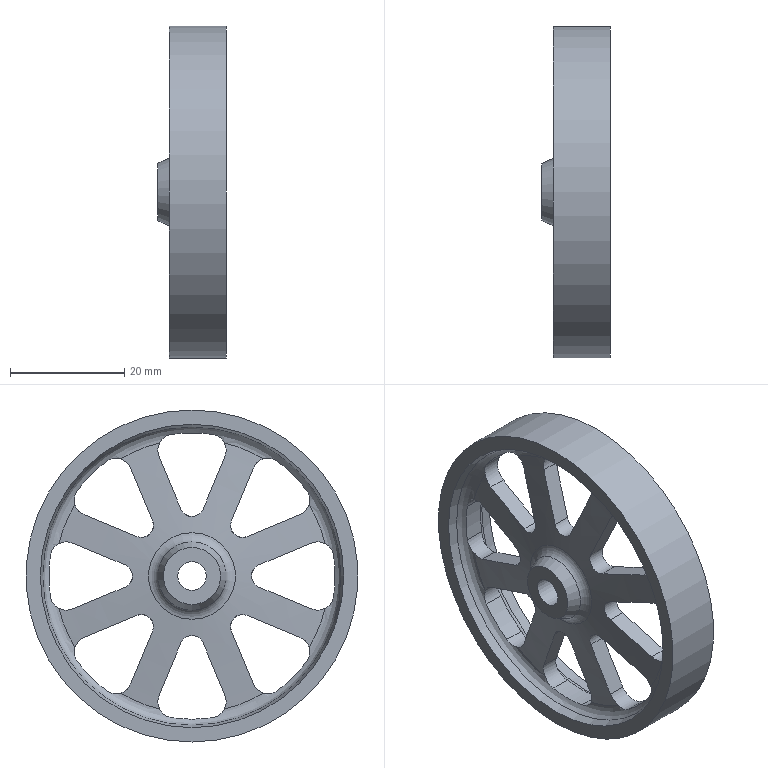Component | NX | WHEEL | 1 solid | 64 faces | volume 9412 mm3 | cylinder 34 | plane 20 | cone 6 | torus 4 | commonest cylinder face diameters 5.6 x16 50 x8 4.2 x8 58 x1 5 x1